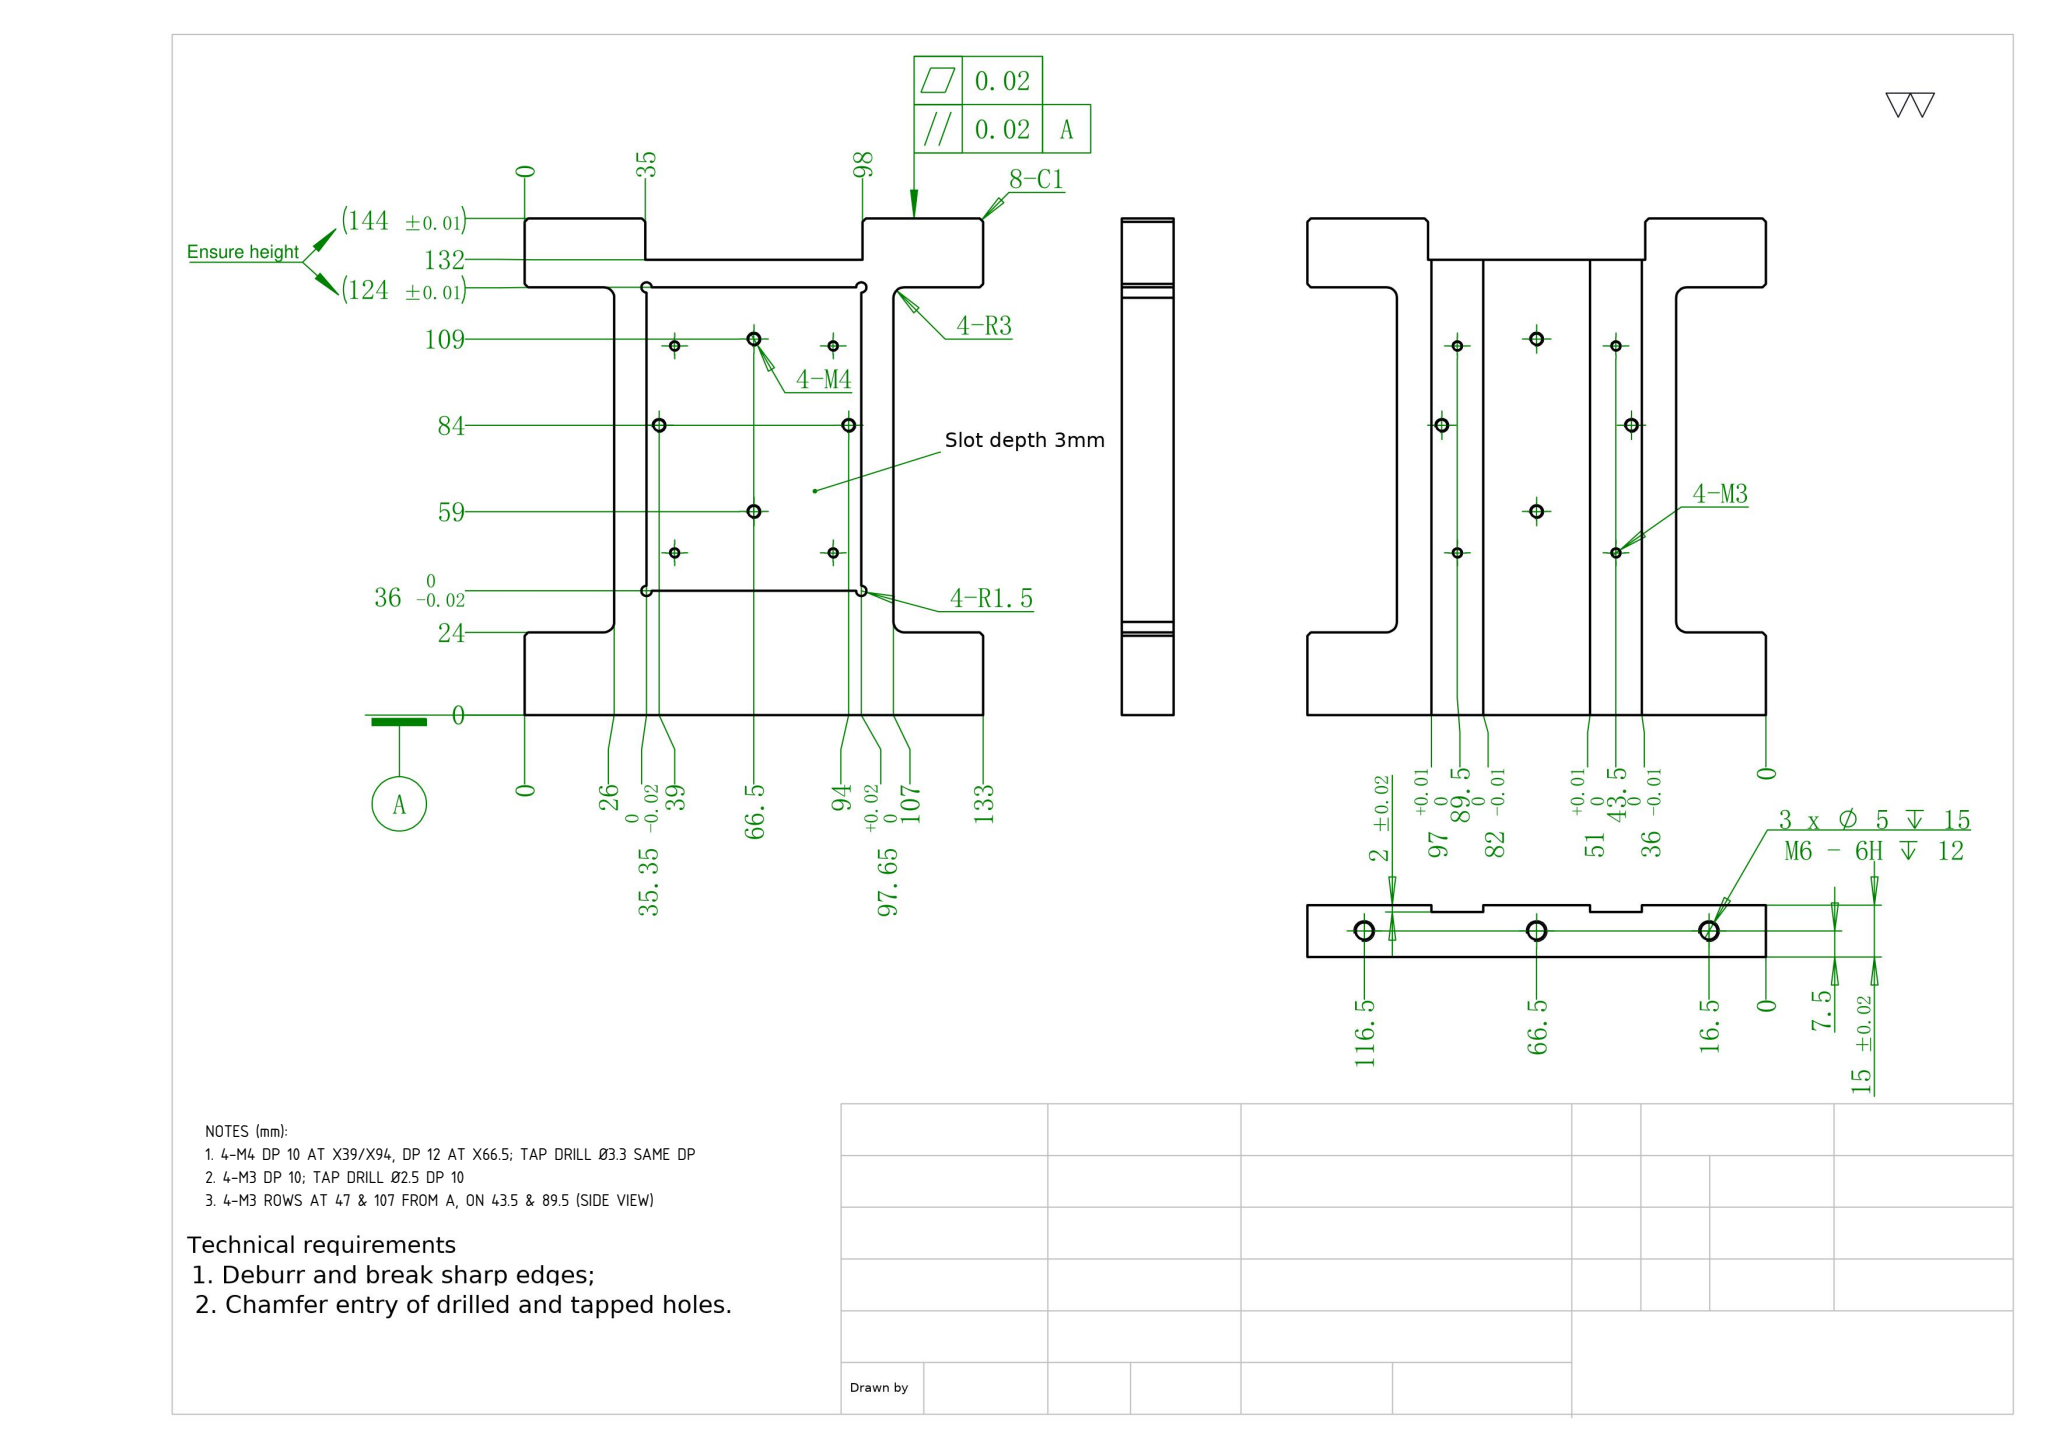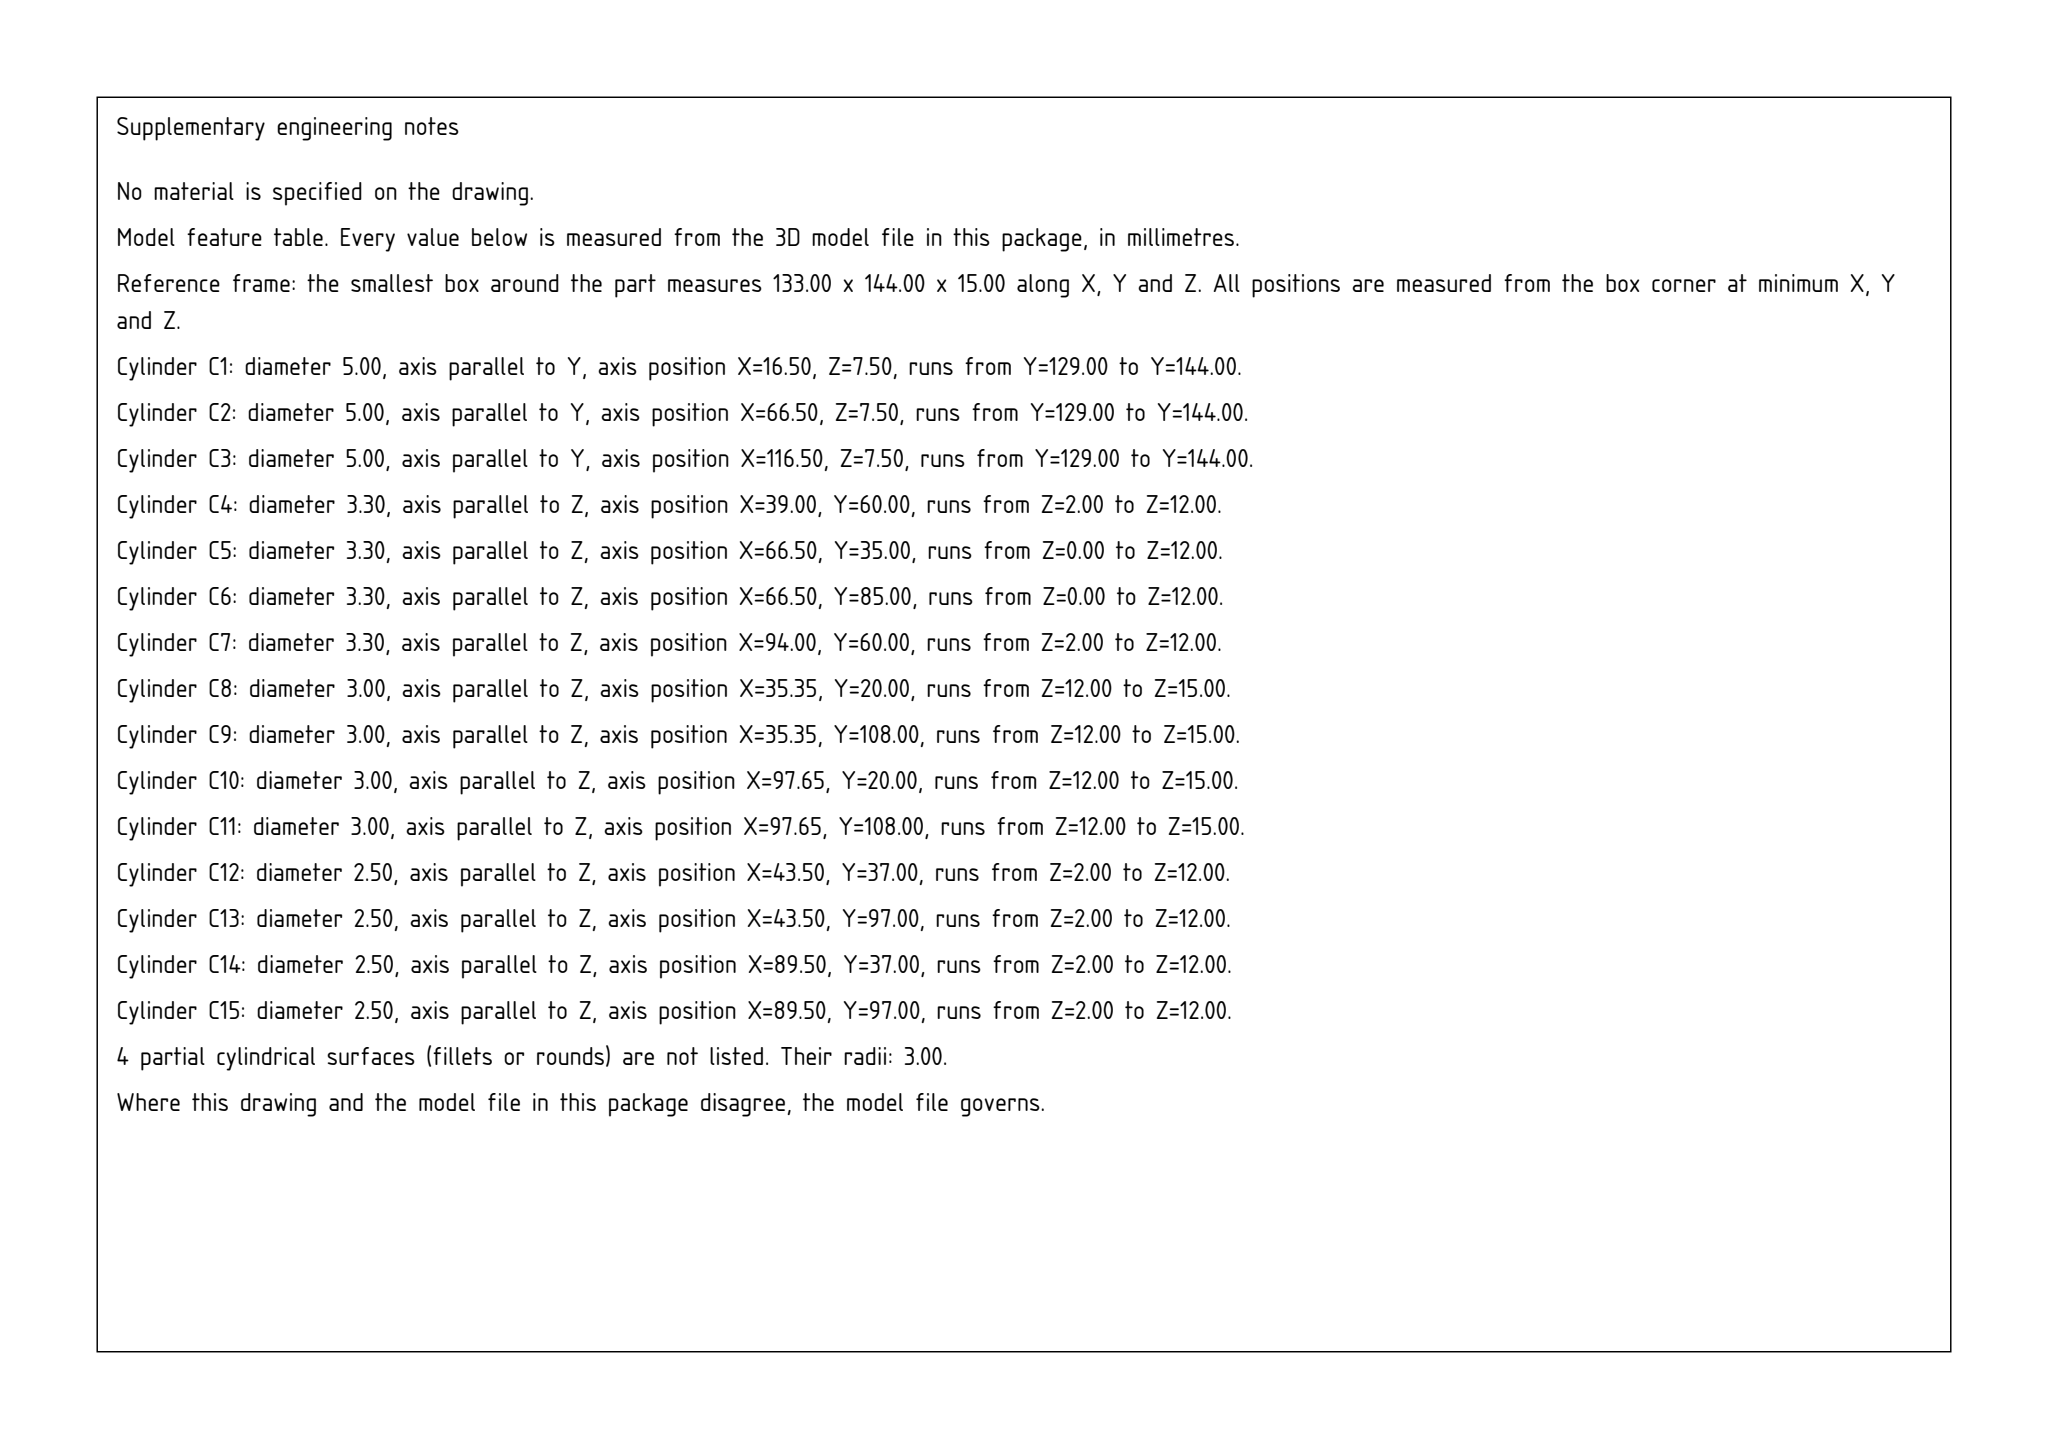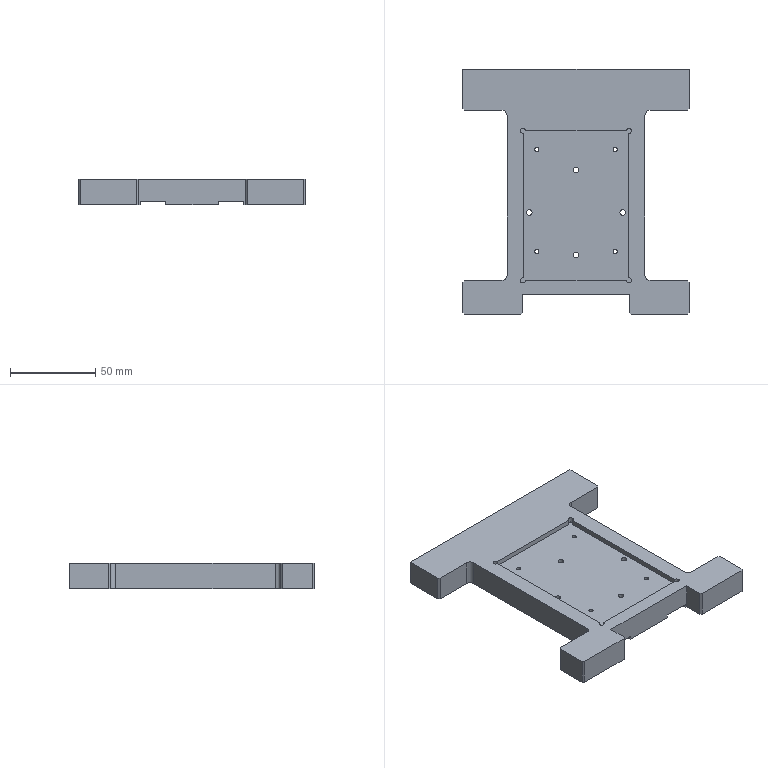Part | SolidWorks | mm | 1 solid | 77 faces | box 133 x 144 x 15 mm | volume 172079 mm3 | plane 39 | cylinder 32 | cone 6 | commonest cylinder face diameters 3.3 x8 2.5 x8 3 x6 5 x6 6 x4
Drawing notes:
4-M4 DP 10 AT X39/X94, DP 12 AT X66.5; TAP DRILL Ø3.3 SAME DP | from the solid: Ø3.3 Z-axis holes: (39,60) & (94,60) len 10; (66.5,35) & (66.5,85) len 12 (M4 tap drill)
4-M3 DP 10; TAP DRILL Ø2.5 DP 10 | from the solid: Ø2.5 Z-axis holes at (43.5,37),(43.5,97),(89.5,37),(89.5,97), len 10 (M3 tap drill)
4-M3 ROWS AT 47 & 107 FROM A, ON 43.5 & 89.5 (SIDE VIEW) | from the solid: Ø2.5 holes z2-12 at (43.5,37),(89.5,37),(43.5,97),(89.5,97); drawing Y=144-y gives rows 107 & 47
build123d program:
from build123d import *

# Parameters (mm, degrees)
SKETCH1_W             = 133
SKETCH1_H             = 132
BOSS_EXTRUDE1_DEPTH   = 15
M6_TAPPED_HOLE1_D     = 5
M6_TAPPED_HOLE1_DEPTH = 15
M6_TAPPED_HOLE1_TIP   = 1.502
M3_TAPPED_HOLE1_D     = 2.5
SKETCH10_W            = 15
SKETCH10_H            = 132
CUT_EXTRUDE3_DEPTH    = 2
SKETCH13_W            = 26
SKETCH13_H            = 100
CUT_EXTRUDE5_DEPTH    = 95.885
SKETCH14_W            = 62.3
SKETCH14_H            = 88
CUT_EXTRUDE6_DEPTH    = 3
SKETCH15_R            = 1.5
CUT_EXTRUDE7_DEPTH    = 3
FILLET1_R             = 3
SKETCH16_W            = 35
SKETCH16_H            = 15
BOSS_EXTRUDE3_DEPTH   = 12
CHAMFER1_SIZE         = 1
M4_TAPPED_HOLE1_D     = 3.3


with BuildPart() as part:
    # Sketch1 → Boss-Extrude1 (new body)
    with BuildSketch(Plane.XY):
        Rectangle(SKETCH1_W, SKETCH1_H)
    extrude(amount=BOSS_EXTRUDE1_DEPTH)

    # M6 Tapped Hole1
    with Locations(Plane(origin=(0, 66, 0), x_dir=(1, 0, 0), z_dir=(0, 1, 0))):
        with Locations((0, -7.5), (-50, -7.5), (50, -7.5)):
            Hole(M6_TAPPED_HOLE1_D / 2, depth=M6_TAPPED_HOLE1_DEPTH)
            with Locations((0, 0, -(M6_TAPPED_HOLE1_DEPTH + M6_TAPPED_HOLE1_TIP / 2))):  # 118° drill point
                Cone(0, M6_TAPPED_HOLE1_D / 2, M6_TAPPED_HOLE1_TIP, mode=Mode.SUBTRACT)

    # M3 Tapped Hole1 (through all)
    with Locations(Plane(origin=(0, 0, 0), x_dir=(-1, 0, 0), z_dir=(0, 0, -1))):
        with Locations((23, -41), (23, 19), (-23, -41), (-23, 19)):
            Hole(M3_TAPPED_HOLE1_D / 2)

    # Sketch10 → Cut-Extrude3 (cut)
    with BuildSketch(Plane(origin=(0, 0, 0), x_dir=(-1, 0, 0), z_dir=(0, 0, -1))):
        with Locations((23, 0)):
            Rectangle(SKETCH10_W, SKETCH10_H)
        with Locations((-23, 0)):
            Rectangle(SKETCH10_W, SKETCH10_H)
    extrude(amount=-CUT_EXTRUDE3_DEPTH, mode=Mode.SUBTRACT)

    # Sketch13 → Cut-Extrude5 (cut, through all)
    with BuildSketch(Plane(origin=(0, 0, 0), x_dir=(-1, 0, 0), z_dir=(0, 0, -1))):
        with Locations((-53.5, -8)):
            Rectangle(SKETCH13_W, SKETCH13_H)
        with Locations((53.5, -8)):
            Rectangle(SKETCH13_W, SKETCH13_H)
    extrude(amount=-CUT_EXTRUDE5_DEPTH, mode=Mode.SUBTRACT)

    # Sketch14 → Cut-Extrude6 (cut)
    with BuildSketch(Plane.XY.offset(15)):
        with Locations((0, -14)):
            Rectangle(SKETCH14_W, SKETCH14_H)
    extrude(amount=-CUT_EXTRUDE6_DEPTH, mode=Mode.SUBTRACT)

    # Sketch15 → Cut-Extrude7 (cut)
    with BuildSketch(Plane.XY.offset(15)):
        with Locations((-31.15, 30)):
            Circle(SKETCH15_R)
        with Locations((31.15, 30)):
            Circle(SKETCH15_R)
        with Locations((31.15, -58)):
            Circle(SKETCH15_R)
        with Locations((-31.15, -58)):
            Circle(SKETCH15_R)
    extrude(amount=-CUT_EXTRUDE7_DEPTH, mode=Mode.SUBTRACT)

    # Fillet1
    fillet1_edges = [part.edges().sort_by_distance(p)[0] for p in [
        (-40.5, -58, 7.5),
        (-40.5, 42, 7.5),
        (40.5, 42, 7.5),
        (40.5, -58, 7.5),
    ]]
    fillet(fillet1_edges, radius=FILLET1_R)

    # Sketch16 → Boss-Extrude3 (add)
    with BuildSketch(Plane.XZ.offset(66)):
        with Locations((49, 7.5)):
            Rectangle(SKETCH16_W, SKETCH16_H)
        with Locations((-49, 7.5)):
            Rectangle(SKETCH16_W, SKETCH16_H)
    extrude(amount=BOSS_EXTRUDE3_DEPTH)

    # Chamfer1
    chamfer1_edges = [part.edges().sort_by_distance(p)[0] for p in [
        (-66.5, -58, 7.5),
        (-66.5, 42, 7.5),
        (66.5, -78, 7.5),
        (31.5, -78, 7.5),
        (-31.5, -78, 7.5),
        (-66.5, -78, 7.5),
        (66.5, -58, 7.5),
        (66.5, 42, 7.5),
    ]]
    chamfer(chamfer1_edges, length=CHAMFER1_SIZE)

    # M4 Tapped Hole1 (through all)
    with Locations(Plane.XY.offset(12)):
        with Locations((0, -43), (27.5, -18), (-27.5, -18), (0, 7)):
            Hole(M4_TAPPED_HOLE1_D / 2)


solid = part.part